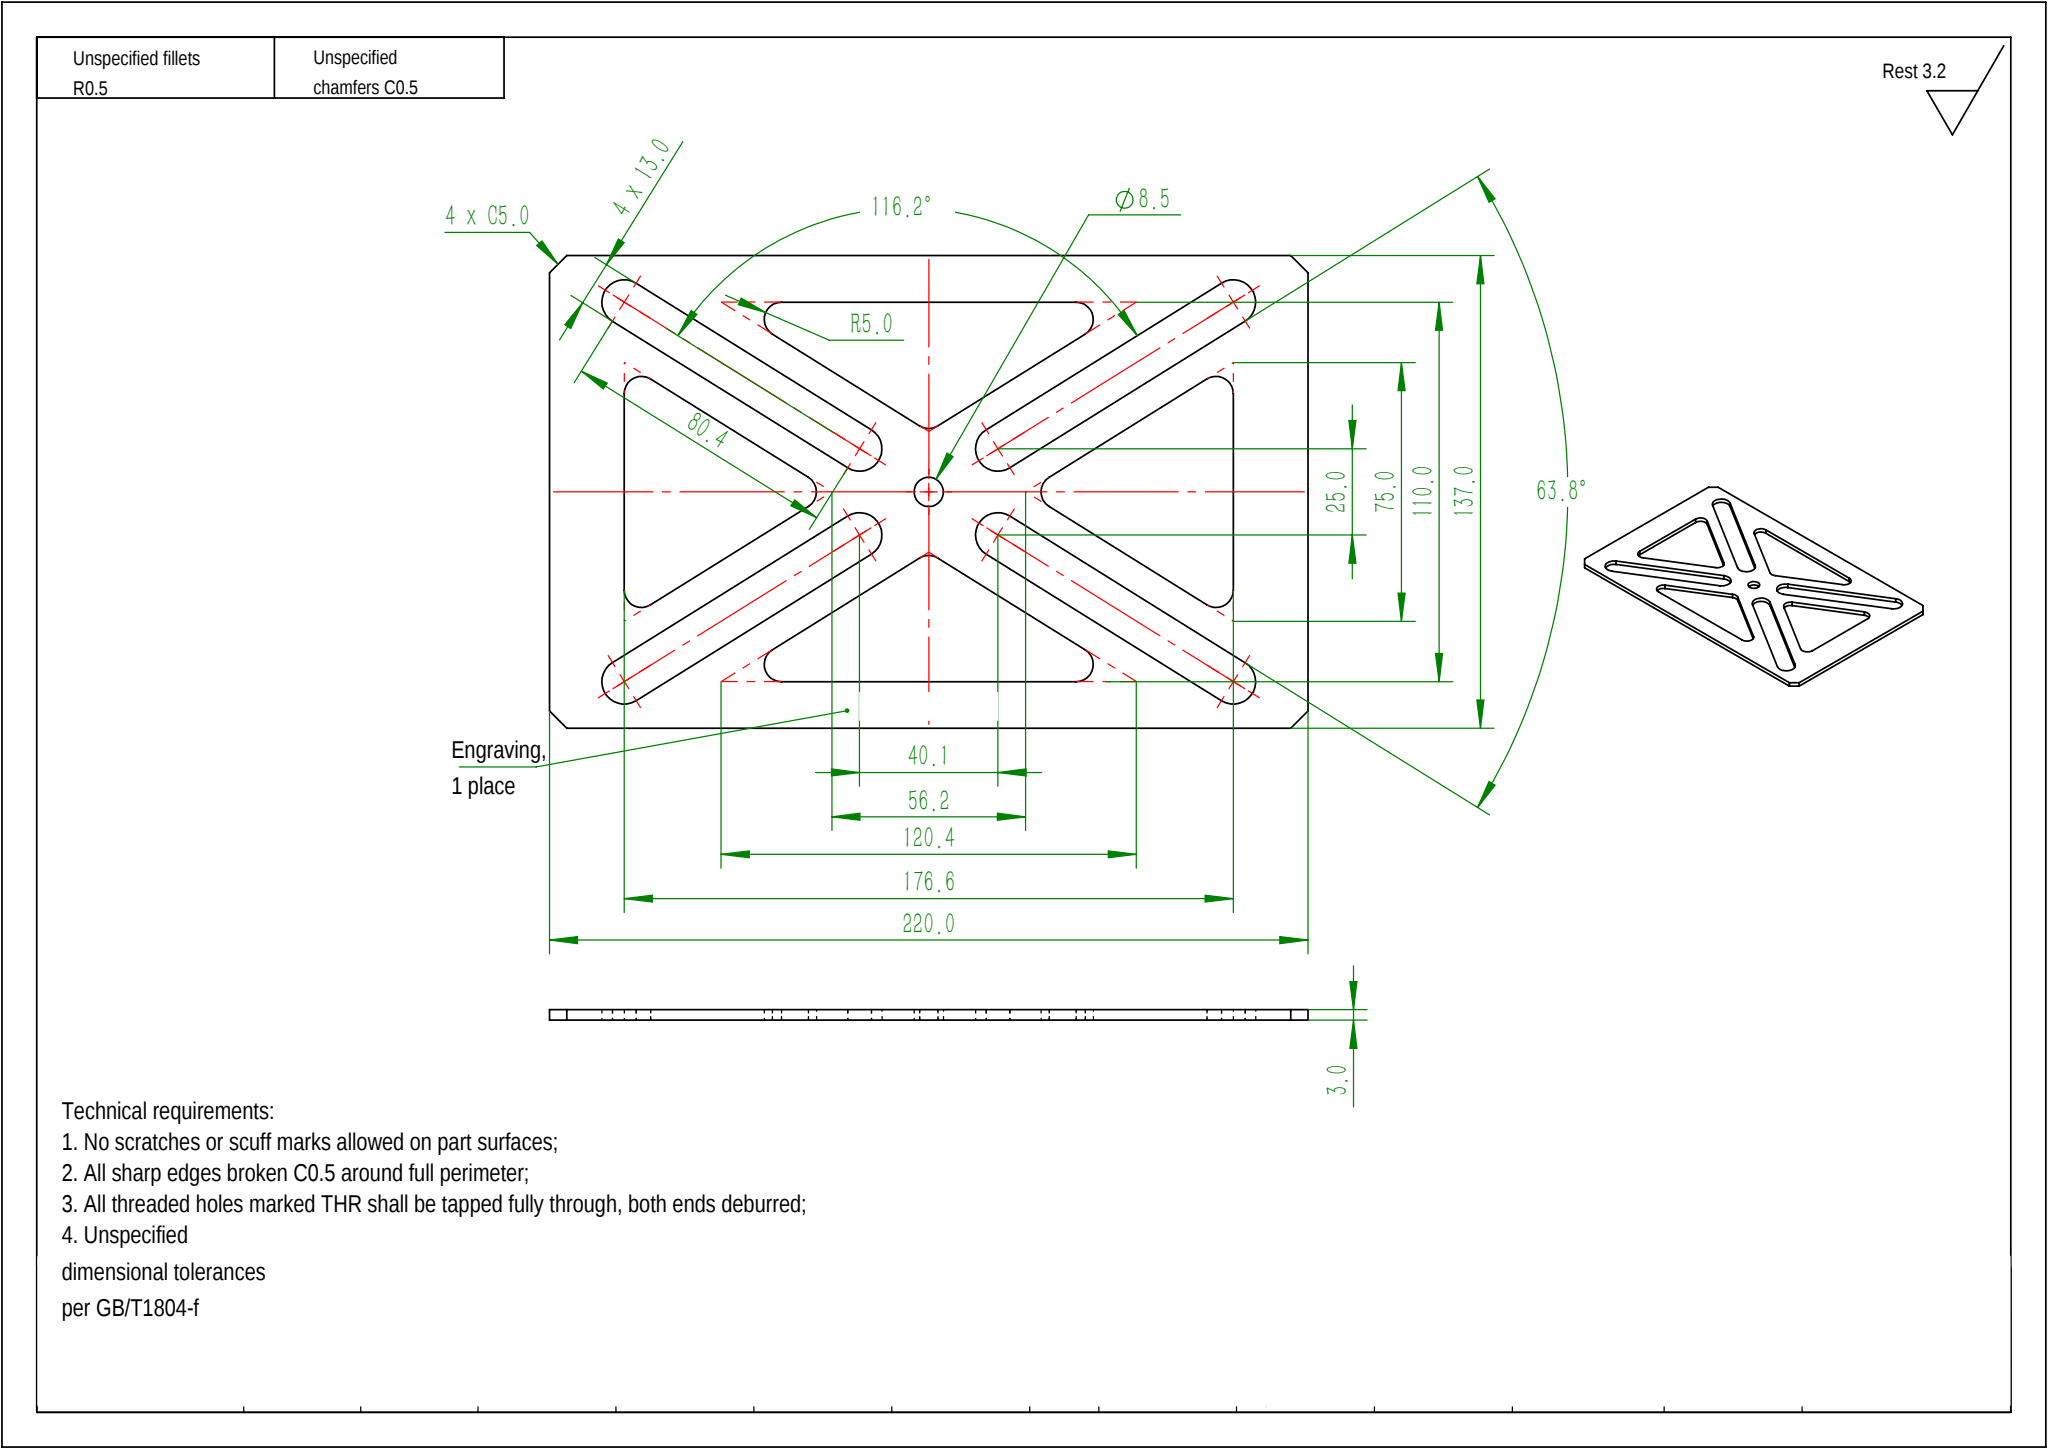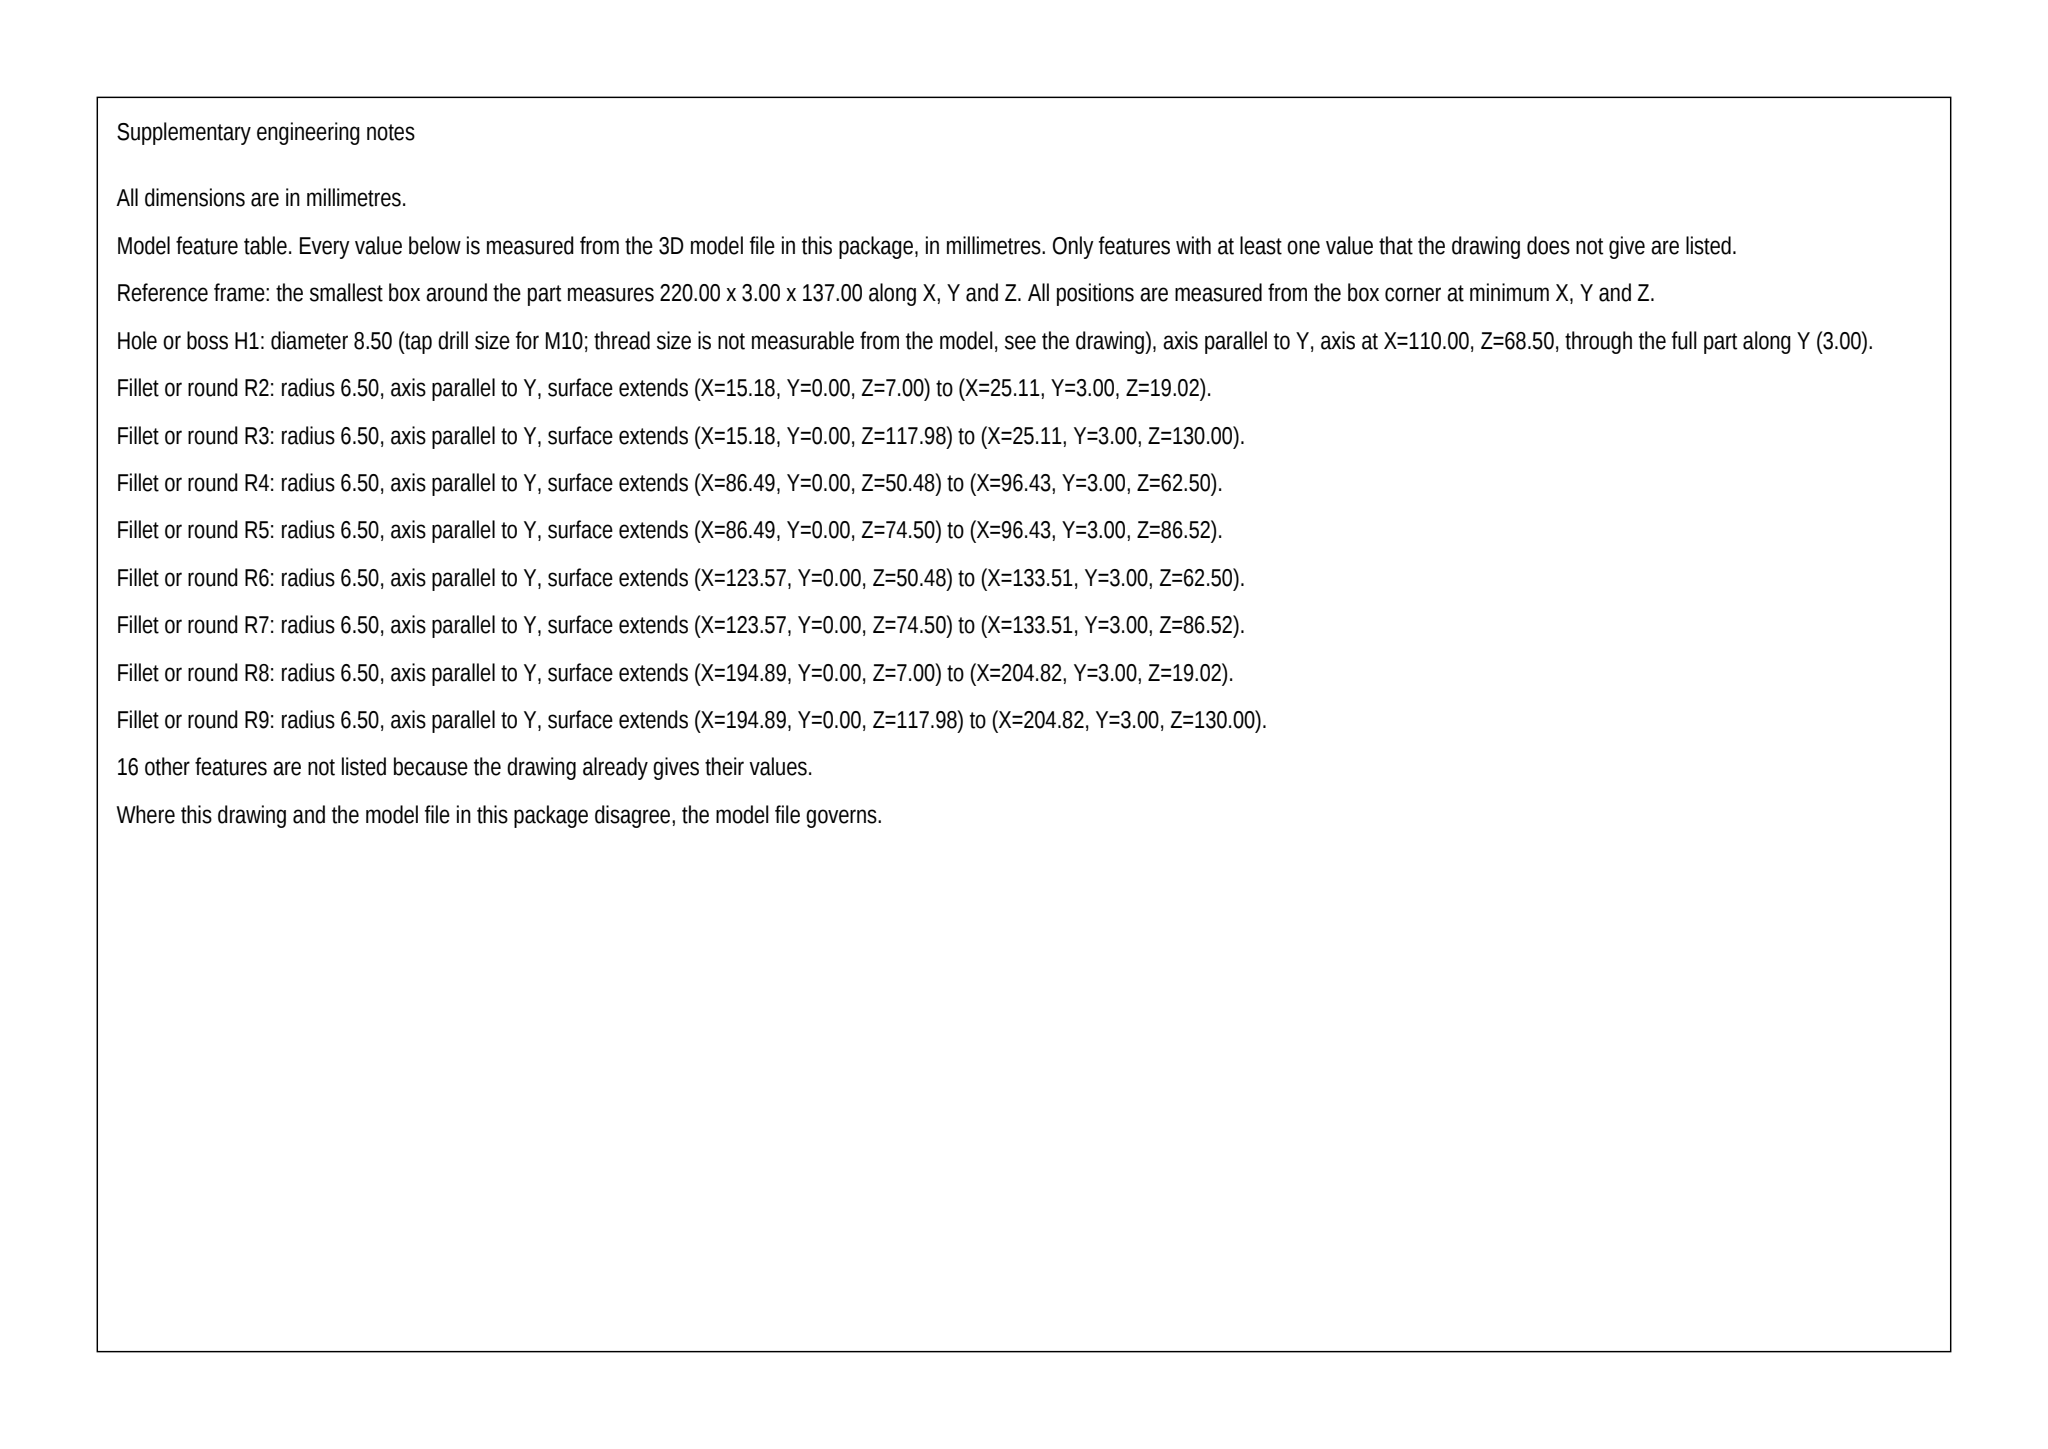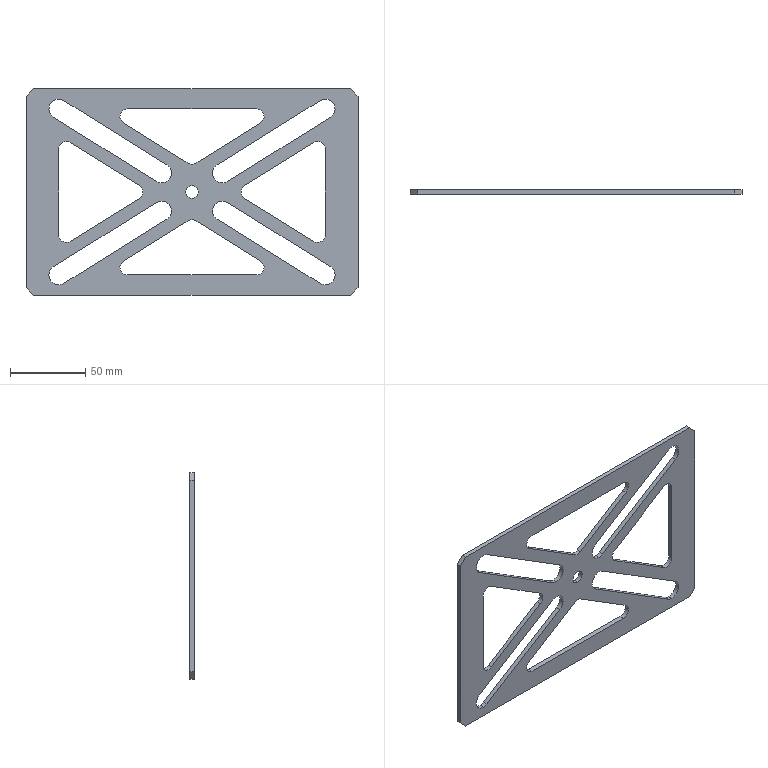Part | SolidWorks | mm | 1 solid | 59 faces | box 220 x 3 x 137 mm | volume 49847 mm3 | plane 30 | cylinder 29 | commonest cylinder face diameters 10 x15 13 x12 8.5 x2
build123d program:
from build123d import *

# Parameters (mm, degrees)
SKETCH1_W                                       = 220
SKETCH1_H                                       = 137
BOSS_EXTRUDE1_DEPTH                             = 8
M8_HEX_SOCKET_HEAD_CAP_SCREW_CBORE1_D           = 9
M8_HEX_SOCKET_HEAD_CAP_SCREW_CBORE1_CBORE_D     = 15
M8_HEX_SOCKET_HEAD_CAP_SCREW_CBORE1_CBORE_DEPTH = 8.6
CUT_EXTRUDE1_DEPTH                              = 130.832
CUT_EXTRUDE2_DEPTH                              = 130.832
FILLET1_R                                       = 5
CHAMFER2_SIZE                                   = 5
CUT_EXTRUDE3_DEPTH                              = 4
BOSS_EXTRUDE3_START                             = -4
SKETCH11_R                                      = 7.5
SKETCH11_R_2                                    = 4.25
BOSS_EXTRUDE3_DEPTH                             = 4
SKETCH12_W                                      = 261.643
SKETCH12_H                                      = 172.285
CUT_EXTRUDE4_DEPTH                              = 5


with BuildPart() as part:
    # Sketch1 → Boss-Extrude1 (new body)
    with BuildSketch(Plane(origin=(0, 0, 0), x_dir=(1, 0, 0), z_dir=(0, 1, 0))):
        Rectangle(SKETCH1_W, SKETCH1_H)
    extrude(amount=BOSS_EXTRUDE1_DEPTH)

    # M8 Hex Socket Head Cap Screw CBORE1 (through all)
    with Locations(Plane(origin=(0, 8, 0), x_dir=(1, 0, 0), z_dir=(0, 1, 0))):
        with Locations((0, 0)):
            CounterBoreHole(M8_HEX_SOCKET_HEAD_CAP_SCREW_CBORE1_D / 2, M8_HEX_SOCKET_HEAD_CAP_SCREW_CBORE1_CBORE_D / 2, M8_HEX_SOCKET_HEAD_CAP_SCREW_CBORE1_CBORE_DEPTH)

    # Sketch5 → Cut-Extrude1 (cut, through all)
    with BuildSketch(Plane(origin=(0, 0, 0), x_dir=(-1, 0, 0), z_dir=(0, -1, 0))):
        with BuildLine():
            Line((84.885, -60.518), (16.637, -18.018))
            ThreePointArc((16.637, -18.018), (14.555, -9.064), (23.509, -6.982))
            Line((23.509, -6.982), (91.757, -49.482))
            ThreePointArc((91.757, -49.482), (93.839, -58.436), (84.885, -60.518))
        make_face()
        with BuildLine():
            Line((-16.637, -18.018), (-84.885, -60.518))
            ThreePointArc((-84.885, -60.518), (-93.839, -58.436), (-91.757, -49.482))
            Line((-91.757, -49.482), (-23.509, -6.982))
            ThreePointArc((-23.509, -6.982), (-14.555, -9.064), (-16.637, -18.018))
        make_face()
        with BuildLine():
            Line((91.757, 49.482), (23.509, 6.982))
            ThreePointArc((23.509, 6.982), (14.555, 9.064), (16.637, 18.018))
            Line((16.637, 18.018), (84.885, 60.518))
            ThreePointArc((84.885, 60.518), (93.839, 58.436), (91.757, 49.482))
        make_face()
        with BuildLine():
            Line((-23.509, 6.982), (-91.757, 49.482))
            ThreePointArc((-91.757, 49.482), (-93.839, 58.436), (-84.885, 60.518))
            Line((-84.885, 60.518), (-16.637, 18.018))
            ThreePointArc((-16.637, 18.018), (-14.555, 9.064), (-23.509, 6.982))
        make_face()
    extrude(amount=-CUT_EXTRUDE1_DEPTH, mode=Mode.SUBTRACT)

    # Sketch6 → Cut-Extrude2 (cut, through all)
    with BuildSketch(Plane.XZ):
        Polygon((0, -17.5), (-60.219, -55), (60.219, -55), align=None)
        Polygon((28.102, 0), (88.321, 37.5), (88.321, -37.5), align=None)
        Polygon((-28.102, 0), (-88.321, 37.5), (-88.321, -37.5), align=None)
        Polygon((0, 17.5), (60.219, 55), (-60.219, 55), align=None)
    extrude(amount=-CUT_EXTRUDE2_DEPTH, mode=Mode.SUBTRACT)

    # Fillet1
    fillet1_edges = [part.edges().sort_by_distance(p)[0] for p in [
        (-28.102, 4, 0),
        (-88.321, 4, -37.5),
        (-88.321, 4, 37.5),
        (0, 4, 17.5),
        (-60.219, 4, 55),
        (60.219, 4, 55),
        (88.321, 4, -37.5),
        (28.102, 4, 0),
        (88.321, 4, 37.5),
        (0, 4, -17.5),
        (60.219, 4, -55),
        (-60.219, 4, -55),
    ]]
    fillet(fillet1_edges, radius=FILLET1_R)

    # Chamfer2
    chamfer2_edges = [part.edges().sort_by_distance(p)[0] for p in [
        (110, 4, 68.5),
        (-110, 4, 68.5),
        (-110, 4, -68.5),
        (110, 4, -68.5),
    ]]
    chamfer(chamfer2_edges, length=CHAMFER2_SIZE)

    # Sketch10 → Cut-Extrude3 (cut)
    with BuildSketch(Plane(origin=(0, 8, 0), x_dir=(1, 0, 0), z_dir=(0, 1, 0))):
        with BuildLine():
            Line((-94.136, -45.662), (-25.888, -3.162))
            ThreePointArc((-25.888, -3.162), (-10.735, -6.685), (-14.258, -21.838))
            Line((-14.258, -21.838), (-82.506, -64.338))
            ThreePointArc((-82.506, -64.338), (-97.659, -60.815), (-94.136, -45.662))
        make_face()
        with BuildLine():
            Line((-25.888, 3.162), (-94.136, 45.662))
            ThreePointArc((-94.136, 45.662), (-97.659, 60.815), (-82.506, 64.338))
            Line((-82.506, 64.338), (-14.258, 21.838))
            ThreePointArc((-14.258, 21.838), (-10.735, 6.685), (-25.888, 3.162))
        make_face()
        with BuildLine():
            Line((14.258, 21.838), (82.506, 64.338))
            ThreePointArc((82.506, 64.338), (97.659, 60.815), (94.136, 45.662))
            Line((94.136, 45.662), (25.888, 3.162))
            ThreePointArc((25.888, 3.162), (10.735, 6.685), (14.258, 21.838))
        make_face()
        with BuildLine():
            Line((24.287, -5.734), (92.535, -48.234))
            ThreePointArc((92.535, -48.234), (95.088, -59.214), (84.108, -61.766))
            Line((84.108, -61.766), (15.859, -19.266))
            ThreePointArc((15.859, -19.266), (13.307, -8.286), (24.287, -5.734))
        make_face()
    extrude(amount=-CUT_EXTRUDE3_DEPTH, mode=Mode.SUBTRACT)

    # Sketch11 → Boss-Extrude3 (add)
    with BuildSketch(Plane.XZ.offset(BOSS_EXTRUDE3_START)):
        with Locations(Location((0, 0, 0), (0, 0, 90))):
            Circle(SKETCH11_R)
        with Locations(Location((0, 0, 0), (0, 0, 270))):
            Circle(SKETCH11_R_2, mode=Mode.SUBTRACT)
    extrude(amount=BOSS_EXTRUDE3_DEPTH)

    # Sketch12 → Cut-Extrude4 (cut)
    with BuildSketch(Plane(origin=(0, 8, 0), x_dir=(1, 0, 0), z_dir=(0, 1, 0))):
        with Locations((3.892, -2.031)):
            Rectangle(SKETCH12_W, SKETCH12_H)
    extrude(amount=-CUT_EXTRUDE4_DEPTH, mode=Mode.SUBTRACT)


solid = part.part